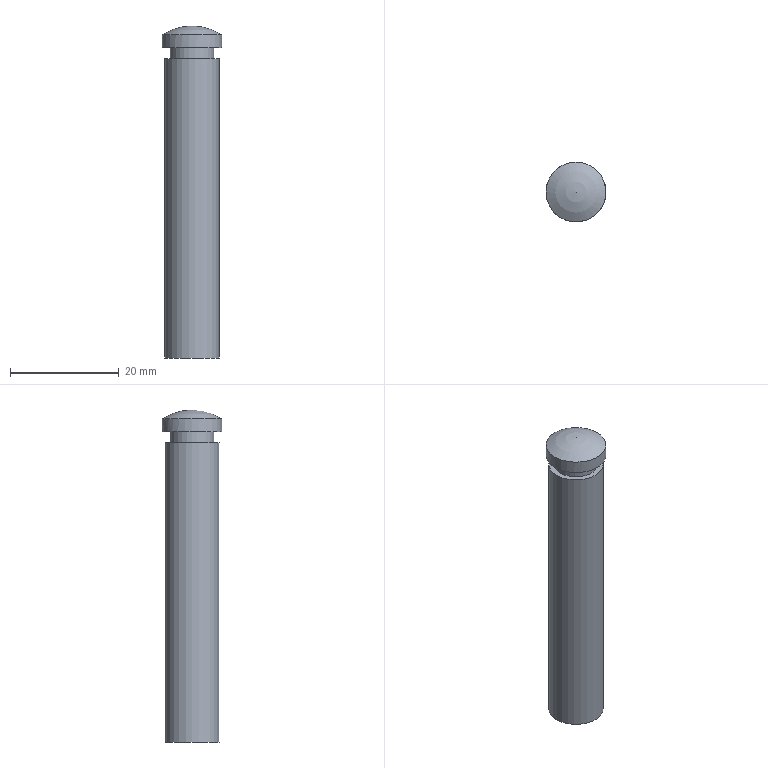Component | NX | SUPPORT_SCREW | 1 solid | 7 faces | box 11 x 11 x 61 mm | volume 4724 mm3 | plane 3 | cylinder 3 | sphere 1 | commonest cylinder face diameters 11 x1 8 x1 10 x1
STEP:
#1=CARTESIAN_POINT('',(0.,0.,0.));
#2=DIRECTION('',(0.,0.,1.));
#3=DIRECTION('',(1.,0.,0.));
#4=AXIS2_PLACEMENT_3D('',#1,#2,#3);
#5=CARTESIAN_POINT('',(-5.,130.,59.));
#6=VERTEX_POINT('',#5);
#7=CARTESIAN_POINT('',(0.,130.,59.));
#8=DIRECTION('',(0.,0.,1.));
#9=DIRECTION('',(-1.,0.,0.));
#10=AXIS2_PLACEMENT_3D('',#7,#8,#9);
#11=CIRCLE('',#10,5.);
#12=CARTESIAN_POINT('',(0.,130.,59.));
#13=DIRECTION('',(0.,0.,1.));
#14=DIRECTION('',(-1.,0.,0.));
#15=AXIS2_PLACEMENT_3D('',#12,#13,#14);
#16=PLANE('',#15);
#17=CARTESIAN_POINT('',(0.,0.));
#18=DIRECTION('',(1.,0.));
#19=AXIS2_PLACEMENT_2D('',#17,#18);
#20=CIRCLE('',#19,5.);
#21=(GEOMETRIC_REPRESENTATION_CONTEXT(2)PARAMETRIC_REPRESENTATION_CONTEXT()REPRESENTATION_CONTEXT('',''));
#22=DEFINITIONAL_REPRESENTATION('',(#20),#21);
#23=PCURVE('',#16,#22);
#24=CARTESIAN_POINT('',(0.,130.,116.));
#25=DIRECTION('',(0.,0.,1.));
#26=DIRECTION('',(-1.,0.,0.));
#27=AXIS2_PLACEMENT_3D('',#24,#25,#26);
#28=CYLINDRICAL_SURFACE('',#27,5.);
#29=CARTESIAN_POINT('',(0.,-57.));
#30=DIRECTION('',(1.,0.));
#31=VECTOR('',#30,1.);
#32=LINE('',#29,#31);
#33=(GEOMETRIC_REPRESENTATION_CONTEXT(2)PARAMETRIC_REPRESENTATION_CONTEXT()REPRESENTATION_CONTEXT('',''));
#34=DEFINITIONAL_REPRESENTATION('',(#32),#33);
#35=PCURVE('',#28,#34);
#36=SURFACE_CURVE('',#11,(#23,#35),.PCURVE_S1.);
#37=EDGE_CURVE('',#6,#6,#36,.T.);
#38=ORIENTED_EDGE('',*,*,#37,.F.);
#39=EDGE_LOOP('',(#38));
#40=FACE_BOUND('',#39,.T.);
#41=ADVANCED_FACE('',(#40),#16,.F.);
#42=CARTESIAN_POINT('',(-5.5,130.,118.352));
#43=VERTEX_POINT('',#42);
#44=CARTESIAN_POINT('',(0.,135.5,118.352));
#45=VERTEX_POINT('',#44);
#46=CARTESIAN_POINT('',(0.,130.,118.352));
#47=DIRECTION('',(0.,0.,1.));
#48=DIRECTION('',(-1.,0.,0.));
#49=AXIS2_PLACEMENT_3D('',#46,#47,#48);
#50=CIRCLE('',#49,5.5);
#51=CARTESIAN_POINT('',(0.,130.,110.));
#52=DIRECTION('',(0.,0.,1.));
#53=DIRECTION('',(0.,1.,0.));
#54=AXIS2_PLACEMENT_3D('',#51,#52,#53);
#55=SPHERICAL_SURFACE('',#54,10.);
#56=CARTESIAN_POINT('',(1.571,0.9884));
#57=CARTESIAN_POINT('',(1.666,0.9884));
#58=CARTESIAN_POINT('',(1.856,0.9884));
#59=CARTESIAN_POINT('',(2.142,0.9884));
#60=CARTESIAN_POINT('',(2.428,0.9884));
#61=CARTESIAN_POINT('',(2.713,0.9884));
#62=CARTESIAN_POINT('',(2.999,0.9884));
#63=CARTESIAN_POINT('',(3.284,0.9884));
#64=CARTESIAN_POINT('',(3.57,0.9884));
#65=CARTESIAN_POINT('',(3.856,0.9884));
#66=CARTESIAN_POINT('',(4.141,0.9884));
#67=CARTESIAN_POINT('',(4.427,0.9884));
#68=CARTESIAN_POINT('',(4.712,0.9884));
#69=CARTESIAN_POINT('',(4.998,0.9884));
#70=CARTESIAN_POINT('',(5.284,0.9884));
#71=CARTESIAN_POINT('',(5.569,0.9884));
#72=CARTESIAN_POINT('',(5.855,0.9884));
#73=CARTESIAN_POINT('',(6.14,0.9884));
#74=CARTESIAN_POINT('',(6.426,0.9884));
#75=CARTESIAN_POINT('',(6.712,0.9884));
#76=CARTESIAN_POINT('',(6.997,0.9884));
#77=CARTESIAN_POINT('',(7.283,0.9884));
#78=CARTESIAN_POINT('',(7.568,0.9884));
#79=CARTESIAN_POINT('',(7.759,0.9884));
#80=CARTESIAN_POINT('',(7.854,0.9884));
#81=B_SPLINE_CURVE_WITH_KNOTS('',3,(#56,#57,#58,#59,#60,#61,#62,#63,#64,#65,#66,#67,#68,#69,#70,#71,#72,#73,#74,#75,#76,#77,#78,#79,#80),.UNSPECIFIED.,.F.,.F.,(4,1,1,1,1,1,1,1,1,1,1,1,1,1,1,1,1,1,1,1,1,1,4),(0.,0.2856,0.5712,0.8568,1.142,1.428,1.714,1.999,2.285,2.57,2.856,3.142,3.427,3.713,3.998,4.284,4.57,4.855,5.141,5.426,5.712,5.998,6.283),.QUASI_UNIFORM_KNOTS.);
#82=(GEOMETRIC_REPRESENTATION_CONTEXT(2)PARAMETRIC_REPRESENTATION_CONTEXT()REPRESENTATION_CONTEXT('',''));
#83=DEFINITIONAL_REPRESENTATION('',(#81),#82);
#84=PCURVE('',#55,#83);
#85=CARTESIAN_POINT('',(0.,130.,116.));
#86=DIRECTION('',(0.,0.,1.));
#87=DIRECTION('',(-1.,0.,0.));
#88=AXIS2_PLACEMENT_3D('',#85,#86,#87);
#89=CYLINDRICAL_SURFACE('',#88,5.5);
#90=CARTESIAN_POINT('',(0.,2.352));
#91=DIRECTION('',(1.,0.));
#92=VECTOR('',#91,1.);
#93=LINE('',#90,#92);
#94=(GEOMETRIC_REPRESENTATION_CONTEXT(2)PARAMETRIC_REPRESENTATION_CONTEXT()REPRESENTATION_CONTEXT('',''));
#95=DEFINITIONAL_REPRESENTATION('',(#93),#94);
#96=PCURVE('',#89,#95);
#97=SURFACE_CURVE('',#50,(#84,#96),.PCURVE_S1.);
#98=EDGE_CURVE('',#43,#45,#97,.T.);
#99=ORIENTED_EDGE('',*,*,#98,.T.);
#100=CARTESIAN_POINT('',(0.,130.,120.));
#101=VERTEX_POINT('',#100);
#102=CARTESIAN_POINT('',(0.,135.5,118.352));
#103=CARTESIAN_POINT('',(0.,134.527,118.992));
#104=CARTESIAN_POINT('',(0.,133.461,119.491));
#105=CARTESIAN_POINT('',(0.,132.329,119.83));
#106=CARTESIAN_POINT('',(0.,131.165,120.));
#107=CARTESIAN_POINT('',(0.,130.,120.));
#108=B_SPLINE_CURVE_WITH_KNOTS('',5,(#102,#103,#104,#105,#106,#107),.UNSPECIFIED.,.F.,.F.,(6,6),(0.9884,1.571),.PIECEWISE_BEZIER_KNOTS.);
#109=CARTESIAN_POINT('',(6.283,0.));
#110=DIRECTION('',(0.,1.));
#111=VECTOR('',#110,1.);
#112=LINE('',#109,#111);
#113=(GEOMETRIC_REPRESENTATION_CONTEXT(2)PARAMETRIC_REPRESENTATION_CONTEXT()REPRESENTATION_CONTEXT('',''));
#114=DEFINITIONAL_REPRESENTATION('',(#112),#113);
#115=PCURVE('',#55,#114);
#116=CARTESIAN_POINT('',(0.,0.));
#117=DIRECTION('',(0.,1.));
#118=VECTOR('',#117,1.);
#119=LINE('',#116,#118);
#120=(GEOMETRIC_REPRESENTATION_CONTEXT(2)PARAMETRIC_REPRESENTATION_CONTEXT()REPRESENTATION_CONTEXT('',''));
#121=DEFINITIONAL_REPRESENTATION('',(#119),#120);
#122=PCURVE('',#55,#121);
#123=SEAM_CURVE('',#108,(#115,#122),.PCURVE_S1.);
#124=EDGE_CURVE('',#45,#101,#123,.T.);
#125=ORIENTED_EDGE('',*,*,#124,.T.);
#126=ORIENTED_EDGE('',*,*,#124,.F.);
#127=CARTESIAN_POINT('',(0.,130.,118.352));
#128=DIRECTION('',(0.,0.,1.));
#129=DIRECTION('',(-1.,0.,0.));
#130=AXIS2_PLACEMENT_3D('',#127,#128,#129);
#131=CIRCLE('',#130,5.5);
#132=CARTESIAN_POINT('',(-4.712,0.9884));
#133=CARTESIAN_POINT('',(-4.617,0.9884));
#134=CARTESIAN_POINT('',(-4.427,0.9884));
#135=CARTESIAN_POINT('',(-4.141,0.9884));
#136=CARTESIAN_POINT('',(-3.856,0.9884));
#137=CARTESIAN_POINT('',(-3.57,0.9884));
#138=CARTESIAN_POINT('',(-3.284,0.9884));
#139=CARTESIAN_POINT('',(-2.999,0.9884));
#140=CARTESIAN_POINT('',(-2.713,0.9884));
#141=CARTESIAN_POINT('',(-2.428,0.9884));
#142=CARTESIAN_POINT('',(-2.142,0.9884));
#143=CARTESIAN_POINT('',(-1.856,0.9884));
#144=CARTESIAN_POINT('',(-1.571,0.9884));
#145=CARTESIAN_POINT('',(-1.285,0.9884));
#146=CARTESIAN_POINT('',(-0.9996,0.9884));
#147=CARTESIAN_POINT('',(-0.714,0.9884));
#148=CARTESIAN_POINT('',(-0.4284,0.9884));
#149=CARTESIAN_POINT('',(-0.1428,0.9884));
#150=CARTESIAN_POINT('',(0.1428,0.9884));
#151=CARTESIAN_POINT('',(0.4284,0.9884));
#152=CARTESIAN_POINT('',(0.714,0.9884));
#153=CARTESIAN_POINT('',(0.9996,0.9884));
#154=CARTESIAN_POINT('',(1.285,0.9884));
#155=CARTESIAN_POINT('',(1.476,0.9884));
#156=CARTESIAN_POINT('',(1.571,0.9884));
#157=B_SPLINE_CURVE_WITH_KNOTS('',3,(#132,#133,#134,#135,#136,#137,#138,#139,#140,#141,#142,#143,#144,#145,#146,#147,#148,#149,#150,#151,#152,#153,#154,#155,#156),.UNSPECIFIED.,.F.,.F.,(4,1,1,1,1,1,1,1,1,1,1,1,1,1,1,1,1,1,1,1,1,1,4),(0.,0.2856,0.5712,0.8568,1.142,1.428,1.714,1.999,2.285,2.57,2.856,3.142,3.427,3.713,3.998,4.284,4.57,4.855,5.141,5.426,5.712,5.998,6.283),.QUASI_UNIFORM_KNOTS.);
#158=(GEOMETRIC_REPRESENTATION_CONTEXT(2)PARAMETRIC_REPRESENTATION_CONTEXT()REPRESENTATION_CONTEXT('',''));
#159=DEFINITIONAL_REPRESENTATION('',(#157),#158);
#160=PCURVE('',#55,#159);
#161=CARTESIAN_POINT('',(0.,2.352));
#162=DIRECTION('',(1.,0.));
#163=VECTOR('',#162,1.);
#164=LINE('',#161,#163);
#165=(GEOMETRIC_REPRESENTATION_CONTEXT(2)PARAMETRIC_REPRESENTATION_CONTEXT()REPRESENTATION_CONTEXT('',''));
#166=DEFINITIONAL_REPRESENTATION('',(#164),#165);
#167=PCURVE('',#89,#166);
#168=SURFACE_CURVE('',#131,(#160,#167),.PCURVE_S1.);
#169=EDGE_CURVE('',#45,#43,#168,.T.);
#170=ORIENTED_EDGE('',*,*,#169,.T.);
#171=EDGE_LOOP('',(#99,#125,#126,#170));
#172=FACE_BOUND('',#171,.T.);
#173=ADVANCED_FACE('',(#172),#55,.T.);
#174=ORIENTED_EDGE('',*,*,#98,.F.);
#175=CARTESIAN_POINT('',(-5.5,130.,116.));
#176=VERTEX_POINT('',#175);
#177=CARTESIAN_POINT('',(-5.5,130.,116.));
#178=CARTESIAN_POINT('',(-5.5,130.,118.352));
#179=B_SPLINE_CURVE_WITH_KNOTS('',1,(#177,#178),.UNSPECIFIED.,.F.,.F.,(2,2),(0.,2.352),.PIECEWISE_BEZIER_KNOTS.);
#180=CARTESIAN_POINT('',(0.,0.));
#181=DIRECTION('',(0.,1.));
#182=VECTOR('',#181,1.);
#183=LINE('',#180,#182);
#184=(GEOMETRIC_REPRESENTATION_CONTEXT(2)PARAMETRIC_REPRESENTATION_CONTEXT()REPRESENTATION_CONTEXT('',''));
#185=DEFINITIONAL_REPRESENTATION('',(#183),#184);
#186=PCURVE('',#89,#185);
#187=CARTESIAN_POINT('',(6.283,0.));
#188=DIRECTION('',(0.,1.));
#189=VECTOR('',#188,1.);
#190=LINE('',#187,#189);
#191=(GEOMETRIC_REPRESENTATION_CONTEXT(2)PARAMETRIC_REPRESENTATION_CONTEXT()REPRESENTATION_CONTEXT('',''));
#192=DEFINITIONAL_REPRESENTATION('',(#190),#191);
#193=PCURVE('',#89,#192);
#194=SEAM_CURVE('',#179,(#186,#193),.PCURVE_S1.);
#195=EDGE_CURVE('',#176,#43,#194,.T.);
#196=ORIENTED_EDGE('',*,*,#195,.F.);
#197=CARTESIAN_POINT('',(0.,130.,116.));
#198=DIRECTION('',(0.,0.,1.));
#199=DIRECTION('',(-1.,0.,0.));
#200=AXIS2_PLACEMENT_3D('',#197,#198,#199);
#201=CIRCLE('',#200,5.5);
#202=CARTESIAN_POINT('',(0.,0.));
#203=DIRECTION('',(1.,0.));
#204=VECTOR('',#203,1.);
#205=LINE('',#202,#204);
#206=(GEOMETRIC_REPRESENTATION_CONTEXT(2)PARAMETRIC_REPRESENTATION_CONTEXT()REPRESENTATION_CONTEXT('',''));
#207=DEFINITIONAL_REPRESENTATION('',(#205),#206);
#208=PCURVE('',#89,#207);
#209=CARTESIAN_POINT('',(0.,134.,116.));
#210=DIRECTION('',(0.,0.,1.));
#211=DIRECTION('',(-1.,0.,0.));
#212=AXIS2_PLACEMENT_3D('',#209,#210,#211);
#213=PLANE('',#212);
#214=CARTESIAN_POINT('',(0.,4.));
#215=DIRECTION('',(1.,0.));
#216=AXIS2_PLACEMENT_2D('',#214,#215);
#217=CIRCLE('',#216,5.5);
#218=(GEOMETRIC_REPRESENTATION_CONTEXT(2)PARAMETRIC_REPRESENTATION_CONTEXT()REPRESENTATION_CONTEXT('',''));
#219=DEFINITIONAL_REPRESENTATION('',(#217),#218);
#220=PCURVE('',#213,#219);
#221=SURFACE_CURVE('',#201,(#208,#220),.PCURVE_S1.);
#222=EDGE_CURVE('',#176,#176,#221,.T.);
#223=ORIENTED_EDGE('',*,*,#222,.T.);
#224=ORIENTED_EDGE('',*,*,#195,.T.);
#225=ORIENTED_EDGE('',*,*,#169,.F.);
#226=EDGE_LOOP('',(#174,#196,#223,#224,#225));
#227=FACE_BOUND('',#226,.T.);
#228=ADVANCED_FACE('',(#227),#89,.T.);
#229=ORIENTED_EDGE('',*,*,#222,.F.);
#230=EDGE_LOOP('',(#229));
#231=FACE_BOUND('',#230,.T.);
#232=CARTESIAN_POINT('',(-4.,130.,116.));
#233=VERTEX_POINT('',#232);
#234=CARTESIAN_POINT('',(0.,130.,116.));
#235=DIRECTION('',(0.,0.,1.));
#236=DIRECTION('',(-1.,0.,0.));
#237=AXIS2_PLACEMENT_3D('',#234,#235,#236);
#238=CIRCLE('',#237,4.);
#239=CARTESIAN_POINT('',(0.,4.));
#240=DIRECTION('',(1.,0.));
#241=AXIS2_PLACEMENT_2D('',#239,#240);
#242=CIRCLE('',#241,4.);
#243=(GEOMETRIC_REPRESENTATION_CONTEXT(2)PARAMETRIC_REPRESENTATION_CONTEXT()REPRESENTATION_CONTEXT('',''));
#244=DEFINITIONAL_REPRESENTATION('',(#242),#243);
#245=PCURVE('',#213,#244);
#246=CARTESIAN_POINT('',(0.,130.,116.));
#247=DIRECTION('',(0.,0.,1.));
#248=DIRECTION('',(-1.,0.,0.));
#249=AXIS2_PLACEMENT_3D('',#246,#247,#248);
#250=CYLINDRICAL_SURFACE('',#249,4.);
#251=CARTESIAN_POINT('',(0.,0.));
#252=DIRECTION('',(1.,0.));
#253=VECTOR('',#252,1.);
#254=LINE('',#251,#253);
#255=(GEOMETRIC_REPRESENTATION_CONTEXT(2)PARAMETRIC_REPRESENTATION_CONTEXT()REPRESENTATION_CONTEXT('',''));
#256=DEFINITIONAL_REPRESENTATION('',(#254),#255);
#257=PCURVE('',#250,#256);
#258=SURFACE_CURVE('',#238,(#245,#257),.PCURVE_S1.);
#259=EDGE_CURVE('',#233,#233,#258,.T.);
#260=ORIENTED_EDGE('',*,*,#259,.T.);
#261=EDGE_LOOP('',(#260));
#262=FACE_BOUND('',#261,.T.);
#263=ADVANCED_FACE('',(#231,#262),#213,.F.);
#264=ORIENTED_EDGE('',*,*,#259,.F.);
#265=CARTESIAN_POINT('',(-4.,130.,114.));
#266=VERTEX_POINT('',#265);
#267=CARTESIAN_POINT('',(-4.,130.,114.));
#268=CARTESIAN_POINT('',(-4.,130.,116.));
#269=B_SPLINE_CURVE_WITH_KNOTS('',1,(#267,#268),.UNSPECIFIED.,.F.,.F.,(2,2),(-2.,0.),.PIECEWISE_BEZIER_KNOTS.);
#270=CARTESIAN_POINT('',(0.,0.));
#271=DIRECTION('',(0.,1.));
#272=VECTOR('',#271,1.);
#273=LINE('',#270,#272);
#274=(GEOMETRIC_REPRESENTATION_CONTEXT(2)PARAMETRIC_REPRESENTATION_CONTEXT()REPRESENTATION_CONTEXT('',''));
#275=DEFINITIONAL_REPRESENTATION('',(#273),#274);
#276=PCURVE('',#250,#275);
#277=CARTESIAN_POINT('',(6.283,0.));
#278=DIRECTION('',(0.,1.));
#279=VECTOR('',#278,1.);
#280=LINE('',#277,#279);
#281=(GEOMETRIC_REPRESENTATION_CONTEXT(2)PARAMETRIC_REPRESENTATION_CONTEXT()REPRESENTATION_CONTEXT('',''));
#282=DEFINITIONAL_REPRESENTATION('',(#280),#281);
#283=PCURVE('',#250,#282);
#284=SEAM_CURVE('',#269,(#276,#283),.PCURVE_S1.);
#285=EDGE_CURVE('',#266,#233,#284,.T.);
#286=ORIENTED_EDGE('',*,*,#285,.F.);
#287=CARTESIAN_POINT('',(0.,130.,114.));
#288=DIRECTION('',(0.,0.,1.));
#289=DIRECTION('',(-1.,0.,0.));
#290=AXIS2_PLACEMENT_3D('',#287,#288,#289);
#291=CIRCLE('',#290,4.);
#292=CARTESIAN_POINT('',(0.,-2.));
#293=DIRECTION('',(1.,0.));
#294=VECTOR('',#293,1.);
#295=LINE('',#292,#294);
#296=(GEOMETRIC_REPRESENTATION_CONTEXT(2)PARAMETRIC_REPRESENTATION_CONTEXT()REPRESENTATION_CONTEXT('',''));
#297=DEFINITIONAL_REPRESENTATION('',(#295),#296);
#298=PCURVE('',#250,#297);
#299=CARTESIAN_POINT('',(0.,135.,114.));
#300=DIRECTION('',(0.,0.,-1.));
#301=DIRECTION('',(1.,0.,0.));
#302=AXIS2_PLACEMENT_3D('',#299,#300,#301);
#303=PLANE('',#302);
#304=CARTESIAN_POINT('',(-4.,5.));
#305=CARTESIAN_POINT('',(-4.,11.928));
#306=CARTESIAN_POINT('',(2.,8.464));
#307=CARTESIAN_POINT('',(8.,5.));
#308=CARTESIAN_POINT('',(2.,1.536));
#309=CARTESIAN_POINT('',(-4.,-1.928));
#310=CARTESIAN_POINT('',(-4.,5.));
#311=(BOUNDED_CURVE()B_SPLINE_CURVE(2,(#304,#305,#306,#307,#308,#309,#310),.UNSPECIFIED.,.T.,.F.)B_SPLINE_CURVE_WITH_KNOTS((1,2,2,2,2,1),(-2.094,0.,2.094,4.189,6.283,8.378),.UNSPECIFIED.)CURVE()GEOMETRIC_REPRESENTATION_ITEM()RATIONAL_B_SPLINE_CURVE((1.,0.5,1.,0.5,1.,0.5,1.))REPRESENTATION_ITEM(''));
#312=(GEOMETRIC_REPRESENTATION_CONTEXT(2)PARAMETRIC_REPRESENTATION_CONTEXT()REPRESENTATION_CONTEXT('',''));
#313=DEFINITIONAL_REPRESENTATION('',(#311),#312);
#314=PCURVE('',#303,#313);
#315=SURFACE_CURVE('',#291,(#298,#314),.PCURVE_S1.);
#316=EDGE_CURVE('',#266,#266,#315,.T.);
#317=ORIENTED_EDGE('',*,*,#316,.T.);
#318=ORIENTED_EDGE('',*,*,#285,.T.);
#319=EDGE_LOOP('',(#264,#286,#317,#318));
#320=FACE_BOUND('',#319,.T.);
#321=ADVANCED_FACE('',(#320),#250,.T.);
#322=ORIENTED_EDGE('',*,*,#316,.F.);
#323=EDGE_LOOP('',(#322));
#324=FACE_BOUND('',#323,.T.);
#325=CARTESIAN_POINT('',(-5.,130.,114.));
#326=VERTEX_POINT('',#325);
#327=CARTESIAN_POINT('',(0.,130.,114.));
#328=DIRECTION('',(0.,0.,1.));
#329=DIRECTION('',(-1.,0.,0.));
#330=AXIS2_PLACEMENT_3D('',#327,#328,#329);
#331=CIRCLE('',#330,5.);
#332=CARTESIAN_POINT('',(-5.,5.));
#333=CARTESIAN_POINT('',(-5.,13.66));
#334=CARTESIAN_POINT('',(2.5,9.33));
#335=CARTESIAN_POINT('',(10.,5.));
#336=CARTESIAN_POINT('',(2.5,0.6699));
#337=CARTESIAN_POINT('',(-5.,-3.66));
#338=CARTESIAN_POINT('',(-5.,5.));
#339=(BOUNDED_CURVE()B_SPLINE_CURVE(2,(#332,#333,#334,#335,#336,#337,#338),.UNSPECIFIED.,.T.,.F.)B_SPLINE_CURVE_WITH_KNOTS((1,2,2,2,2,1),(-2.094,0.,2.094,4.189,6.283,8.378),.UNSPECIFIED.)CURVE()GEOMETRIC_REPRESENTATION_ITEM()RATIONAL_B_SPLINE_CURVE((1.,0.5,1.,0.5,1.,0.5,1.))REPRESENTATION_ITEM(''));
#340=(GEOMETRIC_REPRESENTATION_CONTEXT(2)PARAMETRIC_REPRESENTATION_CONTEXT()REPRESENTATION_CONTEXT('',''));
#341=DEFINITIONAL_REPRESENTATION('',(#339),#340);
#342=PCURVE('',#303,#341);
#343=CARTESIAN_POINT('',(0.,-2.));
#344=DIRECTION('',(1.,0.));
#345=VECTOR('',#344,1.);
#346=LINE('',#343,#345);
#347=(GEOMETRIC_REPRESENTATION_CONTEXT(2)PARAMETRIC_REPRESENTATION_CONTEXT()REPRESENTATION_CONTEXT('',''));
#348=DEFINITIONAL_REPRESENTATION('',(#346),#347);
#349=PCURVE('',#28,#348);
#350=SURFACE_CURVE('',#331,(#342,#349),.PCURVE_S1.);
#351=EDGE_CURVE('',#326,#326,#350,.T.);
#352=ORIENTED_EDGE('',*,*,#351,.T.);
#353=EDGE_LOOP('',(#352));
#354=FACE_BOUND('',#353,.T.);
#355=ADVANCED_FACE('',(#324,#354),#303,.F.);
#356=ORIENTED_EDGE('',*,*,#351,.F.);
#357=CARTESIAN_POINT('',(-5.,130.,59.));
#358=CARTESIAN_POINT('',(-5.,130.,114.));
#359=B_SPLINE_CURVE_WITH_KNOTS('',1,(#357,#358),.UNSPECIFIED.,.F.,.F.,(2,2),(-57.,-2.),.PIECEWISE_BEZIER_KNOTS.);
#360=CARTESIAN_POINT('',(0.,0.));
#361=DIRECTION('',(0.,1.));
#362=VECTOR('',#361,1.);
#363=LINE('',#360,#362);
#364=(GEOMETRIC_REPRESENTATION_CONTEXT(2)PARAMETRIC_REPRESENTATION_CONTEXT()REPRESENTATION_CONTEXT('',''));
#365=DEFINITIONAL_REPRESENTATION('',(#363),#364);
#366=PCURVE('',#28,#365);
#367=CARTESIAN_POINT('',(6.283,0.));
#368=DIRECTION('',(0.,1.));
#369=VECTOR('',#368,1.);
#370=LINE('',#367,#369);
#371=(GEOMETRIC_REPRESENTATION_CONTEXT(2)PARAMETRIC_REPRESENTATION_CONTEXT()REPRESENTATION_CONTEXT('',''));
#372=DEFINITIONAL_REPRESENTATION('',(#370),#371);
#373=PCURVE('',#28,#372);
#374=SEAM_CURVE('',#359,(#366,#373),.PCURVE_S1.);
#375=EDGE_CURVE('',#6,#326,#374,.T.);
#376=ORIENTED_EDGE('',*,*,#375,.F.);
#377=ORIENTED_EDGE('',*,*,#37,.T.);
#378=ORIENTED_EDGE('',*,*,#375,.T.);
#379=EDGE_LOOP('',(#356,#376,#377,#378));
#380=FACE_BOUND('',#379,.T.);
#381=ADVANCED_FACE('',(#380),#28,.T.);
#382=CLOSED_SHELL('',(#41,#173,#228,#263,#321,#355,#381));
#383=MANIFOLD_SOLID_BREP('',#382);
#384=(LENGTH_UNIT()NAMED_UNIT(*)SI_UNIT(.MILLI.,.METRE.));
#385=UNCERTAINTY_MEASURE_WITH_UNIT(LENGTH_MEASURE(0.00001),#384,'','');
#386=(NAMED_UNIT(*)PLANE_ANGLE_UNIT()SI_UNIT($,.RADIAN.));
#387=(NAMED_UNIT(*)SI_UNIT($,.STERADIAN.)SOLID_ANGLE_UNIT());
#388=(GEOMETRIC_REPRESENTATION_CONTEXT(3)GLOBAL_UNCERTAINTY_ASSIGNED_CONTEXT((#385))GLOBAL_UNIT_ASSIGNED_CONTEXT((#384,#386,#387))REPRESENTATION_CONTEXT('',''));
#389=ADVANCED_BREP_SHAPE_REPRESENTATION('',(#4,#383),#388);